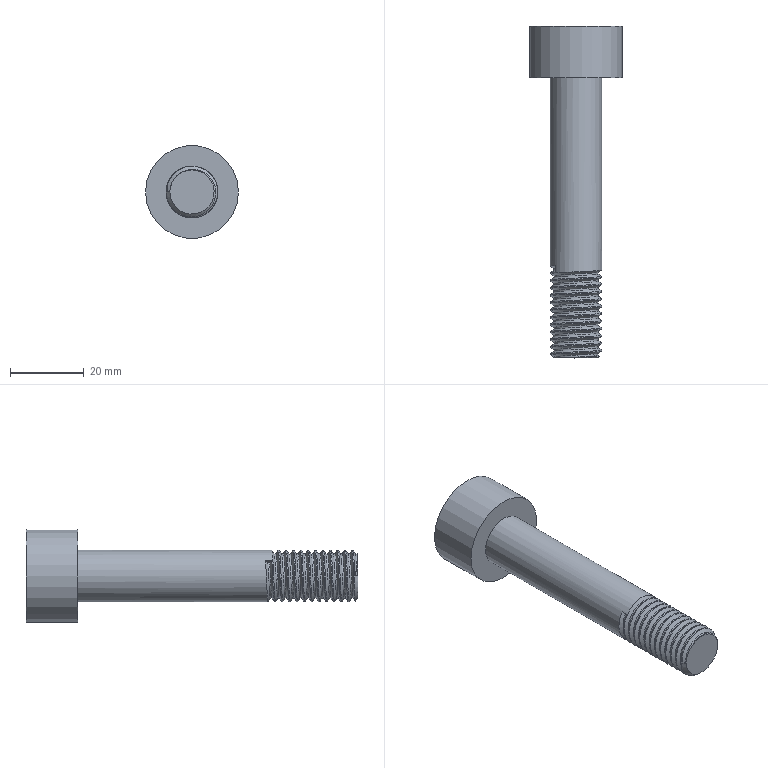Component | NX | ALLINE_SCREW_M14_T_2_PH | 1 solid | 30 faces | volume 17284 mm3 | cylinder 15 | plane 12 | spline 2 | cone 1 | commonest cylinder face diameters 14 x13 25.2 x1 12 x1